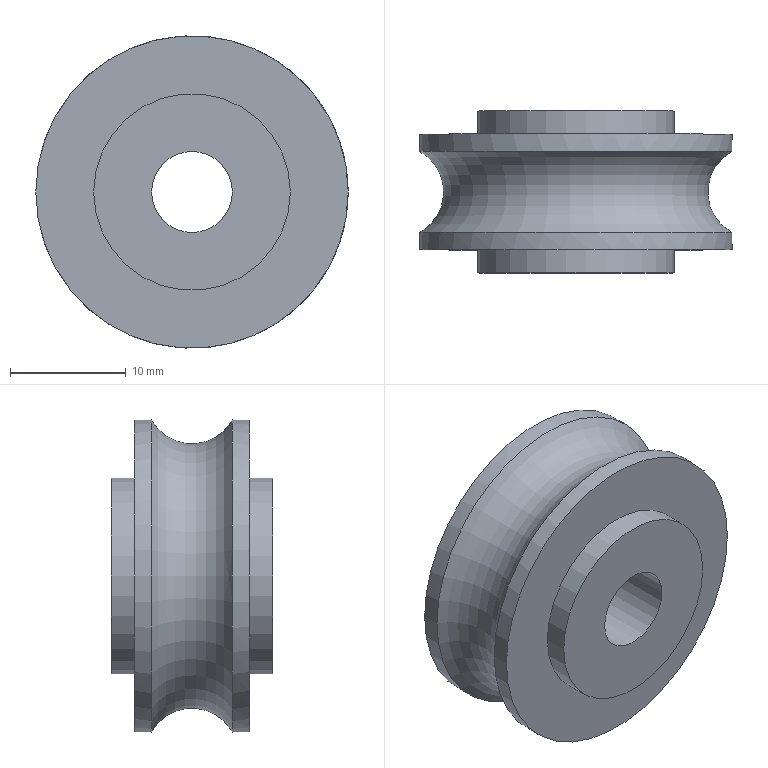Component | NX | PULLEY | 1 solid | 10 faces | box 27 x 14 x 27 mm | volume 5278 mm3 | cylinder 5 | plane 4 | torus 1 | commonest cylinder face diameters 27 x2 17 x2 7 x1
STEP:
#1=CARTESIAN_POINT('',(0.,0.,0.));
#2=DIRECTION('',(0.,0.,1.));
#3=DIRECTION('',(1.,0.,0.));
#4=AXIS2_PLACEMENT_3D('',#1,#2,#3);
#5=CARTESIAN_POINT('',(-13.5,45.5,159.));
#6=VERTEX_POINT('',#5);
#7=CARTESIAN_POINT('',(0.,45.5,159.));
#8=DIRECTION('',(0.,-1.,0.));
#9=DIRECTION('',(-1.,0.,0.));
#10=AXIS2_PLACEMENT_3D('',#7,#8,#9);
#11=CIRCLE('',#10,13.5);
#12=CARTESIAN_POINT('',(0.,44.,159.));
#13=DIRECTION('',(0.,1.,0.));
#14=DIRECTION('',(-1.,0.,0.));
#15=AXIS2_PLACEMENT_3D('',#12,#13,#14);
#16=CYLINDRICAL_SURFACE('',#15,13.5);
#17=CARTESIAN_POINT('',(6.283,1.5));
#18=DIRECTION('',(-1.,0.));
#19=VECTOR('',#18,1.);
#20=LINE('',#17,#19);
#21=(GEOMETRIC_REPRESENTATION_CONTEXT(2)PARAMETRIC_REPRESENTATION_CONTEXT()REPRESENTATION_CONTEXT('',''));
#22=DEFINITIONAL_REPRESENTATION('',(#20),#21);
#23=PCURVE('',#16,#22);
#24=CARTESIAN_POINT('',(0.,49.,159.));
#25=DIRECTION('',(0.,1.,0.));
#26=DIRECTION('',(-1.,0.,0.));
#27=AXIS2_PLACEMENT_3D('',#24,#25,#26);
#28=TOROIDAL_SURFACE('',#27,15.436,4.);
#29=CARTESIAN_POINT('',(6.283,4.207));
#30=DIRECTION('',(-1.,0.));
#31=VECTOR('',#30,1.);
#32=LINE('',#29,#31);
#33=(GEOMETRIC_REPRESENTATION_CONTEXT(2)PARAMETRIC_REPRESENTATION_CONTEXT()REPRESENTATION_CONTEXT('',''));
#34=DEFINITIONAL_REPRESENTATION('',(#32),#33);
#35=PCURVE('',#28,#34);
#36=SURFACE_CURVE('',#11,(#23,#35),.PCURVE_S1.);
#37=EDGE_CURVE('',#6,#6,#36,.T.);
#38=ORIENTED_EDGE('',*,*,#37,.T.);
#39=CARTESIAN_POINT('',(-13.5,44.,159.));
#40=VERTEX_POINT('',#39);
#41=CARTESIAN_POINT('',(-13.5,44.,159.));
#42=CARTESIAN_POINT('',(-13.5,45.5,159.));
#43=B_SPLINE_CURVE_WITH_KNOTS('',1,(#41,#42),.UNSPECIFIED.,.F.,.F.,(2,2),(0.,1.5),.PIECEWISE_BEZIER_KNOTS.);
#44=CARTESIAN_POINT('',(0.,0.));
#45=DIRECTION('',(0.,1.));
#46=VECTOR('',#45,1.);
#47=LINE('',#44,#46);
#48=(GEOMETRIC_REPRESENTATION_CONTEXT(2)PARAMETRIC_REPRESENTATION_CONTEXT()REPRESENTATION_CONTEXT('',''));
#49=DEFINITIONAL_REPRESENTATION('',(#47),#48);
#50=PCURVE('',#16,#49);
#51=CARTESIAN_POINT('',(6.283,0.));
#52=DIRECTION('',(0.,1.));
#53=VECTOR('',#52,1.);
#54=LINE('',#51,#53);
#55=(GEOMETRIC_REPRESENTATION_CONTEXT(2)PARAMETRIC_REPRESENTATION_CONTEXT()REPRESENTATION_CONTEXT('',''));
#56=DEFINITIONAL_REPRESENTATION('',(#54),#55);
#57=PCURVE('',#16,#56);
#58=SEAM_CURVE('',#43,(#50,#57),.PCURVE_S1.);
#59=EDGE_CURVE('',#40,#6,#58,.T.);
#60=ORIENTED_EDGE('',*,*,#59,.F.);
#61=CARTESIAN_POINT('',(13.5,44.,159.));
#62=VERTEX_POINT('',#61);
#63=CARTESIAN_POINT('',(0.,44.,159.));
#64=DIRECTION('',(0.,-1.,0.));
#65=DIRECTION('',(1.,0.,0.));
#66=AXIS2_PLACEMENT_3D('',#63,#64,#65);
#67=CIRCLE('',#66,13.5);
#68=CARTESIAN_POINT('',(3.142,0.));
#69=DIRECTION('',(-1.,0.));
#70=VECTOR('',#69,1.);
#71=LINE('',#68,#70);
#72=(GEOMETRIC_REPRESENTATION_CONTEXT(2)PARAMETRIC_REPRESENTATION_CONTEXT()REPRESENTATION_CONTEXT('',''));
#73=DEFINITIONAL_REPRESENTATION('',(#71),#72);
#74=PCURVE('',#16,#73);
#75=CARTESIAN_POINT('',(0.,44.,159.));
#76=DIRECTION('',(0.,-1.,0.));
#77=DIRECTION('',(1.,0.,0.));
#78=AXIS2_PLACEMENT_3D('',#75,#76,#77);
#79=PLANE('',#78);
#80=CARTESIAN_POINT('',(0.,0.));
#81=DIRECTION('',(1.,0.));
#82=AXIS2_PLACEMENT_2D('',#80,#81);
#83=CIRCLE('',#82,13.5);
#84=(GEOMETRIC_REPRESENTATION_CONTEXT(2)PARAMETRIC_REPRESENTATION_CONTEXT()REPRESENTATION_CONTEXT('',''));
#85=DEFINITIONAL_REPRESENTATION('',(#83),#84);
#86=PCURVE('',#79,#85);
#87=SURFACE_CURVE('',#67,(#74,#86),.PCURVE_S1.);
#88=EDGE_CURVE('',#62,#40,#87,.T.);
#89=ORIENTED_EDGE('',*,*,#88,.F.);
#90=CARTESIAN_POINT('',(0.,44.,159.));
#91=DIRECTION('',(0.,-1.,0.));
#92=DIRECTION('',(1.,0.,0.));
#93=AXIS2_PLACEMENT_3D('',#90,#91,#92);
#94=CIRCLE('',#93,13.5);
#95=CARTESIAN_POINT('',(9.425,0.));
#96=DIRECTION('',(-1.,0.));
#97=VECTOR('',#96,1.);
#98=LINE('',#95,#97);
#99=(GEOMETRIC_REPRESENTATION_CONTEXT(2)PARAMETRIC_REPRESENTATION_CONTEXT()REPRESENTATION_CONTEXT('',''));
#100=DEFINITIONAL_REPRESENTATION('',(#98),#99);
#101=PCURVE('',#16,#100);
#102=CARTESIAN_POINT('',(0.,0.));
#103=DIRECTION('',(1.,0.));
#104=AXIS2_PLACEMENT_2D('',#102,#103);
#105=CIRCLE('',#104,13.5);
#106=(GEOMETRIC_REPRESENTATION_CONTEXT(2)PARAMETRIC_REPRESENTATION_CONTEXT()REPRESENTATION_CONTEXT('',''));
#107=DEFINITIONAL_REPRESENTATION('',(#105),#106);
#108=PCURVE('',#79,#107);
#109=SURFACE_CURVE('',#94,(#101,#108),.PCURVE_S1.);
#110=EDGE_CURVE('',#40,#62,#109,.T.);
#111=ORIENTED_EDGE('',*,*,#110,.F.);
#112=ORIENTED_EDGE('',*,*,#59,.T.);
#113=EDGE_LOOP('',(#38,#60,#89,#111,#112));
#114=FACE_BOUND('',#113,.T.);
#115=ADVANCED_FACE('',(#114),#16,.T.);
#116=CARTESIAN_POINT('',(8.5,44.,159.));
#117=VERTEX_POINT('',#116);
#118=CARTESIAN_POINT('',(0.,44.,159.));
#119=DIRECTION('',(0.,-1.,0.));
#120=DIRECTION('',(1.,0.,0.));
#121=AXIS2_PLACEMENT_3D('',#118,#119,#120);
#122=CIRCLE('',#121,8.5);
#123=CARTESIAN_POINT('',(-0.,0.));
#124=DIRECTION('',(1.,0.));
#125=AXIS2_PLACEMENT_2D('',#123,#124);
#126=CIRCLE('',#125,8.5);
#127=(GEOMETRIC_REPRESENTATION_CONTEXT(2)PARAMETRIC_REPRESENTATION_CONTEXT()REPRESENTATION_CONTEXT('',''));
#128=DEFINITIONAL_REPRESENTATION('',(#126),#127);
#129=PCURVE('',#79,#128);
#130=CARTESIAN_POINT('',(0.,44.,159.));
#131=DIRECTION('',(0.,-1.,0.));
#132=DIRECTION('',(1.,0.,0.));
#133=AXIS2_PLACEMENT_3D('',#130,#131,#132);
#134=CYLINDRICAL_SURFACE('',#133,8.5);
#135=CARTESIAN_POINT('',(0.,0.));
#136=DIRECTION('',(1.,0.));
#137=VECTOR('',#136,1.);
#138=LINE('',#135,#137);
#139=(GEOMETRIC_REPRESENTATION_CONTEXT(2)PARAMETRIC_REPRESENTATION_CONTEXT()REPRESENTATION_CONTEXT('',''));
#140=DEFINITIONAL_REPRESENTATION('',(#138),#139);
#141=PCURVE('',#134,#140);
#142=SURFACE_CURVE('',#122,(#129,#141),.PCURVE_S1.);
#143=EDGE_CURVE('',#117,#117,#142,.T.);
#144=ORIENTED_EDGE('',*,*,#143,.F.);
#145=EDGE_LOOP('',(#144));
#146=FACE_BOUND('',#145,.T.);
#147=ORIENTED_EDGE('',*,*,#88,.T.);
#148=ORIENTED_EDGE('',*,*,#110,.T.);
#149=EDGE_LOOP('',(#147,#148));
#150=FACE_BOUND('',#149,.T.);
#151=ADVANCED_FACE('',(#146,#150),#79,.T.);
#152=CARTESIAN_POINT('',(3.5,42.,159.));
#153=VERTEX_POINT('',#152);
#154=CARTESIAN_POINT('',(0.,42.,159.));
#155=DIRECTION('',(0.,-1.,0.));
#156=DIRECTION('',(1.,0.,0.));
#157=AXIS2_PLACEMENT_3D('',#154,#155,#156);
#158=CIRCLE('',#157,3.5);
#159=CARTESIAN_POINT('',(0.,42.,159.));
#160=DIRECTION('',(0.,-1.,0.));
#161=DIRECTION('',(1.,0.,0.));
#162=AXIS2_PLACEMENT_3D('',#159,#160,#161);
#163=PLANE('',#162);
#164=CARTESIAN_POINT('',(0.,0.));
#165=DIRECTION('',(1.,0.));
#166=AXIS2_PLACEMENT_2D('',#164,#165);
#167=CIRCLE('',#166,3.5);
#168=(GEOMETRIC_REPRESENTATION_CONTEXT(2)PARAMETRIC_REPRESENTATION_CONTEXT()REPRESENTATION_CONTEXT('',''));
#169=DEFINITIONAL_REPRESENTATION('',(#167),#168);
#170=PCURVE('',#163,#169);
#171=CARTESIAN_POINT('',(0.,31.,159.));
#172=DIRECTION('',(0.,1.,0.));
#173=DIRECTION('',(-1.,0.,0.));
#174=AXIS2_PLACEMENT_3D('',#171,#172,#173);
#175=CYLINDRICAL_SURFACE('',#174,3.5);
#176=CARTESIAN_POINT('',(9.425,11.));
#177=DIRECTION('',(-1.,0.));
#178=VECTOR('',#177,1.);
#179=LINE('',#176,#178);
#180=(GEOMETRIC_REPRESENTATION_CONTEXT(2)PARAMETRIC_REPRESENTATION_CONTEXT()REPRESENTATION_CONTEXT('',''));
#181=DEFINITIONAL_REPRESENTATION('',(#179),#180);
#182=PCURVE('',#175,#181);
#183=SURFACE_CURVE('',#158,(#170,#182),.PCURVE_S1.);
#184=EDGE_CURVE('',#153,#153,#183,.T.);
#185=ORIENTED_EDGE('',*,*,#184,.F.);
#186=EDGE_LOOP('',(#185));
#187=FACE_BOUND('',#186,.T.);
#188=CARTESIAN_POINT('',(8.5,42.,159.));
#189=VERTEX_POINT('',#188);
#190=CARTESIAN_POINT('',(0.,42.,159.));
#191=DIRECTION('',(0.,-1.,0.));
#192=DIRECTION('',(1.,0.,0.));
#193=AXIS2_PLACEMENT_3D('',#190,#191,#192);
#194=CIRCLE('',#193,8.5);
#195=CARTESIAN_POINT('',(0.,0.));
#196=DIRECTION('',(1.,0.));
#197=AXIS2_PLACEMENT_2D('',#195,#196);
#198=CIRCLE('',#197,8.5);
#199=(GEOMETRIC_REPRESENTATION_CONTEXT(2)PARAMETRIC_REPRESENTATION_CONTEXT()REPRESENTATION_CONTEXT('',''));
#200=DEFINITIONAL_REPRESENTATION('',(#198),#199);
#201=PCURVE('',#163,#200);
#202=CARTESIAN_POINT('',(0.,2.));
#203=DIRECTION('',(1.,0.));
#204=VECTOR('',#203,1.);
#205=LINE('',#202,#204);
#206=(GEOMETRIC_REPRESENTATION_CONTEXT(2)PARAMETRIC_REPRESENTATION_CONTEXT()REPRESENTATION_CONTEXT('',''));
#207=DEFINITIONAL_REPRESENTATION('',(#205),#206);
#208=PCURVE('',#134,#207);
#209=SURFACE_CURVE('',#194,(#201,#208),.PCURVE_S1.);
#210=EDGE_CURVE('',#189,#189,#209,.T.);
#211=ORIENTED_EDGE('',*,*,#210,.T.);
#212=EDGE_LOOP('',(#211));
#213=FACE_BOUND('',#212,.T.);
#214=ADVANCED_FACE('',(#187,#213),#163,.T.);
#215=ORIENTED_EDGE('',*,*,#210,.F.);
#216=CARTESIAN_POINT('',(8.5,44.,159.));
#217=CARTESIAN_POINT('',(8.5,42.,159.));
#218=B_SPLINE_CURVE_WITH_KNOTS('',1,(#216,#217),.UNSPECIFIED.,.F.,.F.,(2,2),(0.,2.),.PIECEWISE_BEZIER_KNOTS.);
#219=CARTESIAN_POINT('',(0.,0.));
#220=DIRECTION('',(0.,1.));
#221=VECTOR('',#220,1.);
#222=LINE('',#219,#221);
#223=(GEOMETRIC_REPRESENTATION_CONTEXT(2)PARAMETRIC_REPRESENTATION_CONTEXT()REPRESENTATION_CONTEXT('',''));
#224=DEFINITIONAL_REPRESENTATION('',(#222),#223);
#225=PCURVE('',#134,#224);
#226=CARTESIAN_POINT('',(6.283,0.));
#227=DIRECTION('',(0.,1.));
#228=VECTOR('',#227,1.);
#229=LINE('',#226,#228);
#230=(GEOMETRIC_REPRESENTATION_CONTEXT(2)PARAMETRIC_REPRESENTATION_CONTEXT()REPRESENTATION_CONTEXT('',''));
#231=DEFINITIONAL_REPRESENTATION('',(#229),#230);
#232=PCURVE('',#134,#231);
#233=SEAM_CURVE('',#218,(#225,#232),.PCURVE_S1.);
#234=EDGE_CURVE('',#117,#189,#233,.T.);
#235=ORIENTED_EDGE('',*,*,#234,.F.);
#236=ORIENTED_EDGE('',*,*,#143,.T.);
#237=ORIENTED_EDGE('',*,*,#234,.T.);
#238=EDGE_LOOP('',(#215,#235,#236,#237));
#239=FACE_BOUND('',#238,.T.);
#240=ADVANCED_FACE('',(#239),#134,.T.);
#241=CARTESIAN_POINT('',(-13.5,52.5,159.));
#242=VERTEX_POINT('',#241);
#243=CARTESIAN_POINT('',(0.,52.5,159.));
#244=DIRECTION('',(0.,1.,0.));
#245=DIRECTION('',(-1.,0.,0.));
#246=AXIS2_PLACEMENT_3D('',#243,#244,#245);
#247=CIRCLE('',#246,13.5);
#248=CARTESIAN_POINT('',(0.,2.076));
#249=DIRECTION('',(1.,0.));
#250=VECTOR('',#249,1.);
#251=LINE('',#248,#250);
#252=(GEOMETRIC_REPRESENTATION_CONTEXT(2)PARAMETRIC_REPRESENTATION_CONTEXT()REPRESENTATION_CONTEXT('',''));
#253=DEFINITIONAL_REPRESENTATION('',(#251),#252);
#254=PCURVE('',#28,#253);
#255=CARTESIAN_POINT('',(0.,44.,159.));
#256=DIRECTION('',(0.,1.,0.));
#257=DIRECTION('',(-1.,0.,0.));
#258=AXIS2_PLACEMENT_3D('',#255,#256,#257);
#259=CYLINDRICAL_SURFACE('',#258,13.5);
#260=CARTESIAN_POINT('',(0.,8.5));
#261=DIRECTION('',(1.,0.));
#262=VECTOR('',#261,1.);
#263=LINE('',#260,#262);
#264=(GEOMETRIC_REPRESENTATION_CONTEXT(2)PARAMETRIC_REPRESENTATION_CONTEXT()REPRESENTATION_CONTEXT('',''));
#265=DEFINITIONAL_REPRESENTATION('',(#263),#264);
#266=PCURVE('',#259,#265);
#267=SURFACE_CURVE('',#247,(#254,#266),.PCURVE_S1.);
#268=EDGE_CURVE('',#242,#242,#267,.T.);
#269=ORIENTED_EDGE('',*,*,#268,.T.);
#270=CARTESIAN_POINT('',(-13.5,52.5,159.));
#271=CARTESIAN_POINT('',(-12.207,51.785,159.));
#272=CARTESIAN_POINT('',(-11.291,50.543,159.));
#273=CARTESIAN_POINT('',(-10.959,49.,159.));
#274=CARTESIAN_POINT('',(-11.291,47.457,159.));
#275=CARTESIAN_POINT('',(-12.207,46.215,159.));
#276=CARTESIAN_POINT('',(-13.5,45.5,159.));
#277=(BOUNDED_CURVE()B_SPLINE_CURVE(6,(#270,#271,#272,#273,#274,#275,#276),.UNSPECIFIED.,.F.,.F.)B_SPLINE_CURVE_WITH_KNOTS((7,7),(2.076,4.207),.PIECEWISE_BEZIER_KNOTS.)CURVE()GEOMETRIC_REPRESENTATION_ITEM()RATIONAL_B_SPLINE_CURVE((1.059,1.018,0.9962,0.989,0.9962,1.018,1.059))REPRESENTATION_ITEM(''));
#278=CARTESIAN_POINT('',(6.283,0.));
#279=DIRECTION('',(0.,1.));
#280=VECTOR('',#279,1.);
#281=LINE('',#278,#280);
#282=(GEOMETRIC_REPRESENTATION_CONTEXT(2)PARAMETRIC_REPRESENTATION_CONTEXT()REPRESENTATION_CONTEXT('',''));
#283=DEFINITIONAL_REPRESENTATION('',(#281),#282);
#284=PCURVE('',#28,#283);
#285=CARTESIAN_POINT('',(0.,0.));
#286=DIRECTION('',(0.,1.));
#287=VECTOR('',#286,1.);
#288=LINE('',#285,#287);
#289=(GEOMETRIC_REPRESENTATION_CONTEXT(2)PARAMETRIC_REPRESENTATION_CONTEXT()REPRESENTATION_CONTEXT('',''));
#290=DEFINITIONAL_REPRESENTATION('',(#288),#289);
#291=PCURVE('',#28,#290);
#292=SEAM_CURVE('',#277,(#284,#291),.PCURVE_S1.);
#293=EDGE_CURVE('',#242,#6,#292,.T.);
#294=ORIENTED_EDGE('',*,*,#293,.T.);
#295=ORIENTED_EDGE('',*,*,#37,.T.);
#296=ORIENTED_EDGE('',*,*,#293,.F.);
#297=EDGE_LOOP('',(#269,#294,#295,#296));
#298=FACE_BOUND('',#297,.F.);
#299=ADVANCED_FACE('',(#298),#28,.F.);
#300=CARTESIAN_POINT('',(3.5,56.,159.));
#301=VERTEX_POINT('',#300);
#302=CARTESIAN_POINT('',(0.,56.,159.));
#303=DIRECTION('',(0.,1.,0.));
#304=DIRECTION('',(1.,0.,0.));
#305=AXIS2_PLACEMENT_3D('',#302,#303,#304);
#306=CIRCLE('',#305,3.5);
#307=CARTESIAN_POINT('',(0.,56.,159.));
#308=DIRECTION('',(0.,1.,0.));
#309=DIRECTION('',(-1.,0.,0.));
#310=AXIS2_PLACEMENT_3D('',#307,#308,#309);
#311=PLANE('',#310);
#312=CARTESIAN_POINT('',(0.,0.));
#313=DIRECTION('',(-1.,0.));
#314=AXIS2_PLACEMENT_2D('',#312,#313);
#315=CIRCLE('',#314,3.5);
#316=(GEOMETRIC_REPRESENTATION_CONTEXT(2)PARAMETRIC_REPRESENTATION_CONTEXT()REPRESENTATION_CONTEXT('',''));
#317=DEFINITIONAL_REPRESENTATION('',(#315),#316);
#318=PCURVE('',#311,#317);
#319=CARTESIAN_POINT('',(3.142,25.));
#320=DIRECTION('',(1.,0.));
#321=VECTOR('',#320,1.);
#322=LINE('',#319,#321);
#323=(GEOMETRIC_REPRESENTATION_CONTEXT(2)PARAMETRIC_REPRESENTATION_CONTEXT()REPRESENTATION_CONTEXT('',''));
#324=DEFINITIONAL_REPRESENTATION('',(#322),#323);
#325=PCURVE('',#175,#324);
#326=SURFACE_CURVE('',#306,(#318,#325),.PCURVE_S1.);
#327=EDGE_CURVE('',#301,#301,#326,.T.);
#328=ORIENTED_EDGE('',*,*,#327,.F.);
#329=EDGE_LOOP('',(#328));
#330=FACE_BOUND('',#329,.T.);
#331=CARTESIAN_POINT('',(-8.5,56.,159.));
#332=VERTEX_POINT('',#331);
#333=CARTESIAN_POINT('',(0.,56.,159.));
#334=DIRECTION('',(0.,1.,0.));
#335=DIRECTION('',(-1.,0.,0.));
#336=AXIS2_PLACEMENT_3D('',#333,#334,#335);
#337=CIRCLE('',#336,8.5);
#338=CARTESIAN_POINT('',(0.,0.));
#339=DIRECTION('',(1.,0.));
#340=AXIS2_PLACEMENT_2D('',#338,#339);
#341=CIRCLE('',#340,8.5);
#342=(GEOMETRIC_REPRESENTATION_CONTEXT(2)PARAMETRIC_REPRESENTATION_CONTEXT()REPRESENTATION_CONTEXT('',''));
#343=DEFINITIONAL_REPRESENTATION('',(#341),#342);
#344=PCURVE('',#311,#343);
#345=CARTESIAN_POINT('',(0.,54.,159.));
#346=DIRECTION('',(0.,1.,0.));
#347=DIRECTION('',(-1.,0.,0.));
#348=AXIS2_PLACEMENT_3D('',#345,#346,#347);
#349=CYLINDRICAL_SURFACE('',#348,8.5);
#350=CARTESIAN_POINT('',(0.,2.));
#351=DIRECTION('',(1.,0.));
#352=VECTOR('',#351,1.);
#353=LINE('',#350,#352);
#354=(GEOMETRIC_REPRESENTATION_CONTEXT(2)PARAMETRIC_REPRESENTATION_CONTEXT()REPRESENTATION_CONTEXT('',''));
#355=DEFINITIONAL_REPRESENTATION('',(#353),#354);
#356=PCURVE('',#349,#355);
#357=SURFACE_CURVE('',#337,(#344,#356),.PCURVE_S1.);
#358=EDGE_CURVE('',#332,#332,#357,.T.);
#359=ORIENTED_EDGE('',*,*,#358,.T.);
#360=EDGE_LOOP('',(#359));
#361=FACE_BOUND('',#360,.T.);
#362=ADVANCED_FACE('',(#330,#361),#311,.T.);
#363=ORIENTED_EDGE('',*,*,#358,.F.);
#364=CARTESIAN_POINT('',(-8.5,54.,159.));
#365=VERTEX_POINT('',#364);
#366=CARTESIAN_POINT('',(-8.5,54.,159.));
#367=CARTESIAN_POINT('',(-8.5,56.,159.));
#368=B_SPLINE_CURVE_WITH_KNOTS('',1,(#366,#367),.UNSPECIFIED.,.F.,.F.,(2,2),(0.,2.),.PIECEWISE_BEZIER_KNOTS.);
#369=CARTESIAN_POINT('',(0.,0.));
#370=DIRECTION('',(0.,1.));
#371=VECTOR('',#370,1.);
#372=LINE('',#369,#371);
#373=(GEOMETRIC_REPRESENTATION_CONTEXT(2)PARAMETRIC_REPRESENTATION_CONTEXT()REPRESENTATION_CONTEXT('',''));
#374=DEFINITIONAL_REPRESENTATION('',(#372),#373);
#375=PCURVE('',#349,#374);
#376=CARTESIAN_POINT('',(6.283,0.));
#377=DIRECTION('',(0.,1.));
#378=VECTOR('',#377,1.);
#379=LINE('',#376,#378);
#380=(GEOMETRIC_REPRESENTATION_CONTEXT(2)PARAMETRIC_REPRESENTATION_CONTEXT()REPRESENTATION_CONTEXT('',''));
#381=DEFINITIONAL_REPRESENTATION('',(#379),#380);
#382=PCURVE('',#349,#381);
#383=SEAM_CURVE('',#368,(#375,#382),.PCURVE_S1.);
#384=EDGE_CURVE('',#365,#332,#383,.T.);
#385=ORIENTED_EDGE('',*,*,#384,.F.);
#386=CARTESIAN_POINT('',(0.,54.,159.));
#387=DIRECTION('',(0.,1.,0.));
#388=DIRECTION('',(-1.,0.,0.));
#389=AXIS2_PLACEMENT_3D('',#386,#387,#388);
#390=CIRCLE('',#389,8.5);
#391=CARTESIAN_POINT('',(0.,0.));
#392=DIRECTION('',(1.,0.));
#393=VECTOR('',#392,1.);
#394=LINE('',#391,#393);
#395=(GEOMETRIC_REPRESENTATION_CONTEXT(2)PARAMETRIC_REPRESENTATION_CONTEXT()REPRESENTATION_CONTEXT('',''));
#396=DEFINITIONAL_REPRESENTATION('',(#394),#395);
#397=PCURVE('',#349,#396);
#398=CARTESIAN_POINT('',(0.,54.,159.));
#399=DIRECTION('',(0.,-1.,0.));
#400=DIRECTION('',(1.,0.,0.));
#401=AXIS2_PLACEMENT_3D('',#398,#399,#400);
#402=PLANE('',#401);
#403=CARTESIAN_POINT('',(-8.5,0.));
#404=CARTESIAN_POINT('',(-8.5,14.722));
#405=CARTESIAN_POINT('',(4.25,7.361));
#406=CARTESIAN_POINT('',(17.,0.));
#407=CARTESIAN_POINT('',(4.25,-7.361));
#408=CARTESIAN_POINT('',(-8.5,-14.722));
#409=CARTESIAN_POINT('',(-8.5,0.));
#410=(BOUNDED_CURVE()B_SPLINE_CURVE(2,(#403,#404,#405,#406,#407,#408,#409),.UNSPECIFIED.,.T.,.F.)B_SPLINE_CURVE_WITH_KNOTS((1,2,2,2,2,1),(-2.094,0.,2.094,4.189,6.283,8.378),.UNSPECIFIED.)CURVE()GEOMETRIC_REPRESENTATION_ITEM()RATIONAL_B_SPLINE_CURVE((1.,0.5,1.,0.5,1.,0.5,1.))REPRESENTATION_ITEM(''));
#411=(GEOMETRIC_REPRESENTATION_CONTEXT(2)PARAMETRIC_REPRESENTATION_CONTEXT()REPRESENTATION_CONTEXT('',''));
#412=DEFINITIONAL_REPRESENTATION('',(#410),#411);
#413=PCURVE('',#402,#412);
#414=SURFACE_CURVE('',#390,(#397,#413),.PCURVE_S1.);
#415=EDGE_CURVE('',#365,#365,#414,.T.);
#416=ORIENTED_EDGE('',*,*,#415,.T.);
#417=ORIENTED_EDGE('',*,*,#384,.T.);
#418=EDGE_LOOP('',(#363,#385,#416,#417));
#419=FACE_BOUND('',#418,.T.);
#420=ADVANCED_FACE('',(#419),#349,.T.);
#421=ORIENTED_EDGE('',*,*,#415,.F.);
#422=EDGE_LOOP('',(#421));
#423=FACE_BOUND('',#422,.T.);
#424=CARTESIAN_POINT('',(13.5,54.,159.));
#425=VERTEX_POINT('',#424);
#426=CARTESIAN_POINT('',(-13.5,54.,159.));
#427=VERTEX_POINT('',#426);
#428=CARTESIAN_POINT('',(0.,54.,159.));
#429=DIRECTION('',(0.,-1.,0.));
#430=DIRECTION('',(1.,0.,0.));
#431=AXIS2_PLACEMENT_3D('',#428,#429,#430);
#432=CIRCLE('',#431,13.5);
#433=CARTESIAN_POINT('',(0.,0.));
#434=DIRECTION('',(1.,0.));
#435=AXIS2_PLACEMENT_2D('',#433,#434);
#436=CIRCLE('',#435,13.5);
#437=(GEOMETRIC_REPRESENTATION_CONTEXT(2)PARAMETRIC_REPRESENTATION_CONTEXT()REPRESENTATION_CONTEXT('',''));
#438=DEFINITIONAL_REPRESENTATION('',(#436),#437);
#439=PCURVE('',#402,#438);
#440=CARTESIAN_POINT('',(3.142,10.));
#441=DIRECTION('',(-1.,0.));
#442=VECTOR('',#441,1.);
#443=LINE('',#440,#442);
#444=(GEOMETRIC_REPRESENTATION_CONTEXT(2)PARAMETRIC_REPRESENTATION_CONTEXT()REPRESENTATION_CONTEXT('',''));
#445=DEFINITIONAL_REPRESENTATION('',(#443),#444);
#446=PCURVE('',#259,#445);
#447=SURFACE_CURVE('',#432,(#439,#446),.PCURVE_S1.);
#448=EDGE_CURVE('',#425,#427,#447,.T.);
#449=ORIENTED_EDGE('',*,*,#448,.F.);
#450=CARTESIAN_POINT('',(0.,54.,159.));
#451=DIRECTION('',(0.,-1.,0.));
#452=DIRECTION('',(1.,0.,0.));
#453=AXIS2_PLACEMENT_3D('',#450,#451,#452);
#454=CIRCLE('',#453,13.5);
#455=CARTESIAN_POINT('',(0.,0.));
#456=DIRECTION('',(1.,0.));
#457=AXIS2_PLACEMENT_2D('',#455,#456);
#458=CIRCLE('',#457,13.5);
#459=(GEOMETRIC_REPRESENTATION_CONTEXT(2)PARAMETRIC_REPRESENTATION_CONTEXT()REPRESENTATION_CONTEXT('',''));
#460=DEFINITIONAL_REPRESENTATION('',(#458),#459);
#461=PCURVE('',#402,#460);
#462=CARTESIAN_POINT('',(9.425,10.));
#463=DIRECTION('',(-1.,0.));
#464=VECTOR('',#463,1.);
#465=LINE('',#462,#464);
#466=(GEOMETRIC_REPRESENTATION_CONTEXT(2)PARAMETRIC_REPRESENTATION_CONTEXT()REPRESENTATION_CONTEXT('',''));
#467=DEFINITIONAL_REPRESENTATION('',(#465),#466);
#468=PCURVE('',#259,#467);
#469=SURFACE_CURVE('',#454,(#461,#468),.PCURVE_S1.);
#470=EDGE_CURVE('',#427,#425,#469,.T.);
#471=ORIENTED_EDGE('',*,*,#470,.F.);
#472=EDGE_LOOP('',(#449,#471));
#473=FACE_BOUND('',#472,.T.);
#474=ADVANCED_FACE('',(#423,#473),#402,.F.);
#475=ORIENTED_EDGE('',*,*,#268,.T.);
#476=CARTESIAN_POINT('',(-13.5,52.5,159.));
#477=CARTESIAN_POINT('',(-13.5,54.,159.));
#478=B_SPLINE_CURVE_WITH_KNOTS('',1,(#476,#477),.UNSPECIFIED.,.F.,.F.,(2,2),(8.5,10.),.PIECEWISE_BEZIER_KNOTS.);
#479=CARTESIAN_POINT('',(6.283,0.));
#480=DIRECTION('',(0.,1.));
#481=VECTOR('',#480,1.);
#482=LINE('',#479,#481);
#483=(GEOMETRIC_REPRESENTATION_CONTEXT(2)PARAMETRIC_REPRESENTATION_CONTEXT()REPRESENTATION_CONTEXT('',''));
#484=DEFINITIONAL_REPRESENTATION('',(#482),#483);
#485=PCURVE('',#259,#484);
#486=CARTESIAN_POINT('',(0.,0.));
#487=DIRECTION('',(0.,1.));
#488=VECTOR('',#487,1.);
#489=LINE('',#486,#488);
#490=(GEOMETRIC_REPRESENTATION_CONTEXT(2)PARAMETRIC_REPRESENTATION_CONTEXT()REPRESENTATION_CONTEXT('',''));
#491=DEFINITIONAL_REPRESENTATION('',(#489),#490);
#492=PCURVE('',#259,#491);
#493=SEAM_CURVE('',#478,(#485,#492),.PCURVE_S1.);
#494=EDGE_CURVE('',#242,#427,#493,.T.);
#495=ORIENTED_EDGE('',*,*,#494,.T.);
#496=ORIENTED_EDGE('',*,*,#470,.T.);
#497=ORIENTED_EDGE('',*,*,#448,.T.);
#498=ORIENTED_EDGE('',*,*,#494,.F.);
#499=EDGE_LOOP('',(#475,#495,#496,#497,#498));
#500=FACE_BOUND('',#499,.T.);
#501=ADVANCED_FACE('',(#500),#259,.T.);
#502=ORIENTED_EDGE('',*,*,#184,.F.);
#503=CARTESIAN_POINT('',(3.5,42.,159.));
#504=CARTESIAN_POINT('',(3.5,56.,159.));
#505=B_SPLINE_CURVE_WITH_KNOTS('',1,(#503,#504),.UNSPECIFIED.,.F.,.F.,(2,2),(11.,25.),.PIECEWISE_BEZIER_KNOTS.);
#506=CARTESIAN_POINT('',(9.425,0.));
#507=DIRECTION('',(0.,1.));
#508=VECTOR('',#507,1.);
#509=LINE('',#506,#508);
#510=(GEOMETRIC_REPRESENTATION_CONTEXT(2)PARAMETRIC_REPRESENTATION_CONTEXT()REPRESENTATION_CONTEXT('',''));
#511=DEFINITIONAL_REPRESENTATION('',(#509),#510);
#512=PCURVE('',#175,#511);
#513=CARTESIAN_POINT('',(3.142,0.));
#514=DIRECTION('',(0.,1.));
#515=VECTOR('',#514,1.);
#516=LINE('',#513,#515);
#517=(GEOMETRIC_REPRESENTATION_CONTEXT(2)PARAMETRIC_REPRESENTATION_CONTEXT()REPRESENTATION_CONTEXT('',''));
#518=DEFINITIONAL_REPRESENTATION('',(#516),#517);
#519=PCURVE('',#175,#518);
#520=SEAM_CURVE('',#505,(#512,#519),.PCURVE_S1.);
#521=EDGE_CURVE('',#153,#301,#520,.T.);
#522=ORIENTED_EDGE('',*,*,#521,.T.);
#523=ORIENTED_EDGE('',*,*,#327,.F.);
#524=ORIENTED_EDGE('',*,*,#521,.F.);
#525=EDGE_LOOP('',(#502,#522,#523,#524));
#526=FACE_BOUND('',#525,.F.);
#527=ADVANCED_FACE('',(#526),#175,.F.);
#528=CLOSED_SHELL('',(#115,#151,#214,#240,#299,#362,#420,#474,#501,#527));
#529=MANIFOLD_SOLID_BREP('',#528);
#530=(LENGTH_UNIT()NAMED_UNIT(*)SI_UNIT(.MILLI.,.METRE.));
#531=UNCERTAINTY_MEASURE_WITH_UNIT(LENGTH_MEASURE(0.000005),#530,'','');
#532=(NAMED_UNIT(*)PLANE_ANGLE_UNIT()SI_UNIT($,.RADIAN.));
#533=(NAMED_UNIT(*)SI_UNIT($,.STERADIAN.)SOLID_ANGLE_UNIT());
#534=(GEOMETRIC_REPRESENTATION_CONTEXT(3)GLOBAL_UNCERTAINTY_ASSIGNED_CONTEXT((#531))GLOBAL_UNIT_ASSIGNED_CONTEXT((#530,#532,#533))REPRESENTATION_CONTEXT('',''));
#535=ADVANCED_BREP_SHAPE_REPRESENTATION('',(#4,#529),#534);